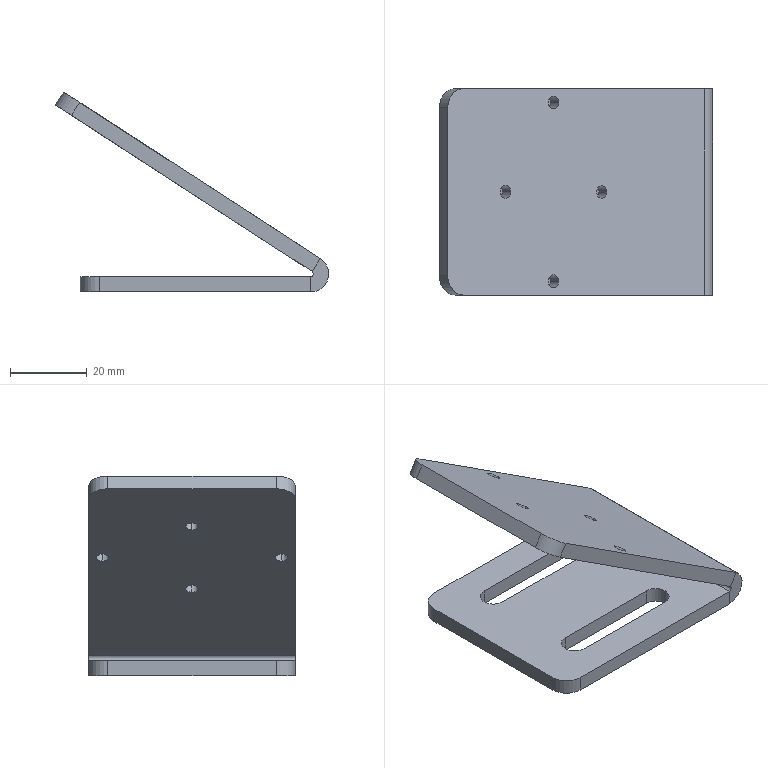Component | SolidWorks | AdjustmentPlate-1 | 1 solid | 34 faces | box 71.44 x 54 x 52.29 mm | volume 29585 mm3 | cylinder 18 | plane 16 | commonest cylinder face diameters 3.3 x8 7 x4 10 x4 9.473 x1 1.473 x1
STEP:
#1=CARTESIAN_POINT('',(2.616,-0.009211,10.905));
#2=VERTEX_POINT('',#1);
#3=CARTESIAN_POINT('',(2.507,-0.009211,10.976));
#4=VERTEX_POINT('',#3);
#5=CARTESIAN_POINT('',(2.562,-0.009211,10.941));
#6=DIRECTION('',(-0.5446,0.,-0.8387));
#7=DIRECTION('',(-0.8387,0.,0.5446));
#8=AXIS2_PLACEMENT_3D('',#5,#6,#7);
#9=CIRCLE('',#8,0.06496);
#10=EDGE_CURVE('',#2,#4,#9,.T.);
#11=ORIENTED_EDGE('',*,*,#10,.T.);
#12=CARTESIAN_POINT('',(2.593,-0.009211,11.108));
#13=VERTEX_POINT('',#12);
#14=CARTESIAN_POINT('',(2.593,-0.009211,11.108));
#15=DIRECTION('',(0.5446,-0.,0.8387));
#16=VECTOR('',#15,39.37);
#17=LINE('',#14,#16);
#18=EDGE_CURVE('',#4,#13,#17,.T.);
#19=ORIENTED_EDGE('',*,*,#18,.T.);
#20=CARTESIAN_POINT('',(2.702,-0.009211,11.037));
#21=VERTEX_POINT('',#20);
#22=CARTESIAN_POINT('',(2.647,-0.009211,11.073));
#23=DIRECTION('',(0.5446,-0.,0.8387));
#24=DIRECTION('',(0.8387,-0.,-0.5446));
#25=AXIS2_PLACEMENT_3D('',#22,#23,#24);
#26=CIRCLE('',#25,0.06496);
#27=EDGE_CURVE('',#13,#21,#26,.T.);
#28=ORIENTED_EDGE('',*,*,#27,.T.);
#29=CARTESIAN_POINT('',(2.702,-0.009211,11.037));
#30=DIRECTION('',(0.5446,-0.,0.8387));
#31=VECTOR('',#30,39.37);
#32=LINE('',#29,#31);
#33=EDGE_CURVE('',#2,#21,#32,.T.);
#34=ORIENTED_EDGE('',*,*,#33,.F.);
#35=EDGE_LOOP('',(#11,#19,#28,#34));
#36=FACE_OUTER_BOUND('',#35,.T.);
#37=CARTESIAN_POINT('',(2.647,-0.009211,11.073));
#38=DIRECTION('',(0.5446,-0.,0.8387));
#39=DIRECTION('',(0.8387,-0.,-0.5446));
#40=AXIS2_PLACEMENT_3D('',#37,#38,#39);
#41=CYLINDRICAL_SURFACE('',#40,0.06496);
#42=ADVANCED_FACE('',(#36),#41,.F.);
#43=CARTESIAN_POINT('',(1.626,-0.009211,11.549));
#44=VERTEX_POINT('',#43);
#45=CARTESIAN_POINT('',(1.517,-0.009211,11.619));
#46=VERTEX_POINT('',#45);
#47=CARTESIAN_POINT('',(1.571,-0.009211,11.584));
#48=DIRECTION('',(-0.5446,0.,-0.8387));
#49=DIRECTION('',(-0.8387,0.,0.5446));
#50=AXIS2_PLACEMENT_3D('',#47,#48,#49);
#51=CIRCLE('',#50,0.06496);
#52=EDGE_CURVE('',#44,#46,#51,.T.);
#53=ORIENTED_EDGE('',*,*,#52,.T.);
#54=CARTESIAN_POINT('',(1.602,-0.009211,11.751));
#55=VERTEX_POINT('',#54);
#56=CARTESIAN_POINT('',(1.602,-0.009211,11.751));
#57=DIRECTION('',(0.5446,-0.,0.8387));
#58=VECTOR('',#57,39.37);
#59=LINE('',#56,#58);
#60=EDGE_CURVE('',#46,#55,#59,.T.);
#61=ORIENTED_EDGE('',*,*,#60,.T.);
#62=CARTESIAN_POINT('',(1.711,-0.009211,11.681));
#63=VERTEX_POINT('',#62);
#64=CARTESIAN_POINT('',(1.657,-0.009211,11.716));
#65=DIRECTION('',(0.5446,-0.,0.8387));
#66=DIRECTION('',(0.8387,-0.,-0.5446));
#67=AXIS2_PLACEMENT_3D('',#64,#65,#66);
#68=CIRCLE('',#67,0.06496);
#69=EDGE_CURVE('',#55,#63,#68,.T.);
#70=ORIENTED_EDGE('',*,*,#69,.T.);
#71=CARTESIAN_POINT('',(1.711,-0.009211,11.681));
#72=DIRECTION('',(0.5446,-0.,0.8387));
#73=VECTOR('',#72,39.37);
#74=LINE('',#71,#73);
#75=EDGE_CURVE('',#44,#63,#74,.T.);
#76=ORIENTED_EDGE('',*,*,#75,.F.);
#77=EDGE_LOOP('',(#53,#61,#70,#76));
#78=FACE_OUTER_BOUND('',#77,.T.);
#79=CARTESIAN_POINT('',(1.657,-0.009211,11.716));
#80=DIRECTION('',(0.5446,-0.,0.8387));
#81=DIRECTION('',(0.8387,-0.,-0.5446));
#82=AXIS2_PLACEMENT_3D('',#79,#80,#81);
#83=CYLINDRICAL_SURFACE('',#82,0.06496);
#84=ADVANCED_FACE('',(#78),#83,.F.);
#85=CARTESIAN_POINT('',(2.121,0.9101,11.227));
#86=VERTEX_POINT('',#85);
#87=CARTESIAN_POINT('',(2.012,0.9101,11.298));
#88=VERTEX_POINT('',#87);
#89=CARTESIAN_POINT('',(2.066,0.9101,11.262));
#90=DIRECTION('',(-0.5446,0.,-0.8387));
#91=DIRECTION('',(-0.8387,0.,0.5446));
#92=AXIS2_PLACEMENT_3D('',#89,#90,#91);
#93=CIRCLE('',#92,0.06496);
#94=EDGE_CURVE('',#86,#88,#93,.T.);
#95=ORIENTED_EDGE('',*,*,#94,.T.);
#96=CARTESIAN_POINT('',(2.098,0.9101,11.43));
#97=VERTEX_POINT('',#96);
#98=CARTESIAN_POINT('',(2.098,0.9101,11.43));
#99=DIRECTION('',(0.5446,-0.,0.8387));
#100=VECTOR('',#99,39.37);
#101=LINE('',#98,#100);
#102=EDGE_CURVE('',#88,#97,#101,.T.);
#103=ORIENTED_EDGE('',*,*,#102,.T.);
#104=CARTESIAN_POINT('',(2.207,0.9101,11.359));
#105=VERTEX_POINT('',#104);
#106=CARTESIAN_POINT('',(2.152,0.9101,11.394));
#107=DIRECTION('',(0.5446,-0.,0.8387));
#108=DIRECTION('',(0.8387,0.,-0.5446));
#109=AXIS2_PLACEMENT_3D('',#106,#107,#108);
#110=CIRCLE('',#109,0.06496);
#111=EDGE_CURVE('',#97,#105,#110,.T.);
#112=ORIENTED_EDGE('',*,*,#111,.T.);
#113=CARTESIAN_POINT('',(2.207,0.9101,11.359));
#114=DIRECTION('',(0.5446,-0.,0.8387));
#115=VECTOR('',#114,39.37);
#116=LINE('',#113,#115);
#117=EDGE_CURVE('',#86,#105,#116,.T.);
#118=ORIENTED_EDGE('',*,*,#117,.F.);
#119=EDGE_LOOP('',(#95,#103,#112,#118));
#120=FACE_OUTER_BOUND('',#119,.T.);
#121=CARTESIAN_POINT('',(2.152,0.9101,11.394));
#122=DIRECTION('',(0.5446,-0.,0.8387));
#123=DIRECTION('',(0.8387,0.,-0.5446));
#124=AXIS2_PLACEMENT_3D('',#121,#122,#123);
#125=CYLINDRICAL_SURFACE('',#124,0.06496);
#126=ADVANCED_FACE('',(#120),#125,.F.);
#127=CARTESIAN_POINT('',(2.121,-0.9285,11.227));
#128=VERTEX_POINT('',#127);
#129=CARTESIAN_POINT('',(2.012,-0.9285,11.298));
#130=VERTEX_POINT('',#129);
#131=CARTESIAN_POINT('',(2.066,-0.9285,11.262));
#132=DIRECTION('',(-0.5446,0.,-0.8387));
#133=DIRECTION('',(-0.8387,0.,0.5446));
#134=AXIS2_PLACEMENT_3D('',#131,#132,#133);
#135=CIRCLE('',#134,0.06496);
#136=EDGE_CURVE('',#128,#130,#135,.T.);
#137=ORIENTED_EDGE('',*,*,#136,.T.);
#138=CARTESIAN_POINT('',(2.098,-0.9285,11.43));
#139=VERTEX_POINT('',#138);
#140=CARTESIAN_POINT('',(2.098,-0.9285,11.43));
#141=DIRECTION('',(0.5446,-0.,0.8387));
#142=VECTOR('',#141,39.37);
#143=LINE('',#140,#142);
#144=EDGE_CURVE('',#130,#139,#143,.T.);
#145=ORIENTED_EDGE('',*,*,#144,.T.);
#146=CARTESIAN_POINT('',(2.207,-0.9285,11.359));
#147=VERTEX_POINT('',#146);
#148=CARTESIAN_POINT('',(2.152,-0.9285,11.394));
#149=DIRECTION('',(0.5446,-0.,0.8387));
#150=DIRECTION('',(0.8387,0.,-0.5446));
#151=AXIS2_PLACEMENT_3D('',#148,#149,#150);
#152=CIRCLE('',#151,0.06496);
#153=EDGE_CURVE('',#139,#147,#152,.T.);
#154=ORIENTED_EDGE('',*,*,#153,.T.);
#155=CARTESIAN_POINT('',(2.207,-0.9285,11.359));
#156=DIRECTION('',(0.5446,-0.,0.8387));
#157=VECTOR('',#156,39.37);
#158=LINE('',#155,#157);
#159=EDGE_CURVE('',#128,#147,#158,.T.);
#160=ORIENTED_EDGE('',*,*,#159,.F.);
#161=EDGE_LOOP('',(#137,#145,#154,#160));
#162=FACE_OUTER_BOUND('',#161,.T.);
#163=CARTESIAN_POINT('',(2.152,-0.9285,11.394));
#164=DIRECTION('',(0.5446,-0.,0.8387));
#165=DIRECTION('',(0.8387,0.,-0.5446));
#166=AXIS2_PLACEMENT_3D('',#163,#164,#165);
#167=CYLINDRICAL_SURFACE('',#166,0.06496);
#168=ADVANCED_FACE('',(#162),#167,.F.);
#169=CARTESIAN_POINT('',(3.006,0.7191,10.043));
#170=VERTEX_POINT('',#169);
#171=CARTESIAN_POINT('',(3.006,0.4435,10.043));
#172=VERTEX_POINT('',#171);
#173=CARTESIAN_POINT('',(3.006,0.5813,10.043));
#174=DIRECTION('',(-0.,-0.,-1.));
#175=DIRECTION('',(0.,1.,0.));
#176=AXIS2_PLACEMENT_3D('',#173,#174,#175);
#177=CIRCLE('',#176,0.1378);
#178=EDGE_CURVE('',#170,#172,#177,.T.);
#179=ORIENTED_EDGE('',*,*,#178,.F.);
#180=CARTESIAN_POINT('',(1.824,0.7191,10.043));
#181=VERTEX_POINT('',#180);
#182=CARTESIAN_POINT('',(2.612,0.7191,10.043));
#183=DIRECTION('',(1.,-0.,-0.));
#184=VECTOR('',#183,39.37);
#185=LINE('',#182,#184);
#186=EDGE_CURVE('',#181,#170,#185,.T.);
#187=ORIENTED_EDGE('',*,*,#186,.F.);
#188=CARTESIAN_POINT('',(1.824,0.4435,10.043));
#189=VERTEX_POINT('',#188);
#190=CARTESIAN_POINT('',(1.824,0.5813,10.043));
#191=DIRECTION('',(-0.,-0.,-1.));
#192=DIRECTION('',(0.,1.,0.));
#193=AXIS2_PLACEMENT_3D('',#190,#191,#192);
#194=CIRCLE('',#193,0.1378);
#195=EDGE_CURVE('',#189,#181,#194,.T.);
#196=ORIENTED_EDGE('',*,*,#195,.F.);
#197=CARTESIAN_POINT('',(2.612,0.4435,10.043));
#198=DIRECTION('',(-1.,0.,0.));
#199=VECTOR('',#198,39.37);
#200=LINE('',#197,#199);
#201=EDGE_CURVE('',#172,#189,#200,.T.);
#202=ORIENTED_EDGE('',*,*,#201,.F.);
#203=EDGE_LOOP('',(#179,#187,#196,#202));
#204=FACE_BOUND('',#203,.T.);
#205=CARTESIAN_POINT('',(1.824,-0.7376,10.043));
#206=VERTEX_POINT('',#205);
#207=CARTESIAN_POINT('',(3.006,-0.7376,10.043));
#208=VERTEX_POINT('',#207);
#209=CARTESIAN_POINT('',(2.612,-0.7376,10.043));
#210=DIRECTION('',(1.,-0.,-0.));
#211=VECTOR('',#210,39.37);
#212=LINE('',#209,#211);
#213=EDGE_CURVE('',#206,#208,#212,.T.);
#214=ORIENTED_EDGE('',*,*,#213,.T.);
#215=CARTESIAN_POINT('',(3.006,-0.462,10.043));
#216=VERTEX_POINT('',#215);
#217=CARTESIAN_POINT('',(3.006,-0.5998,10.043));
#218=DIRECTION('',(0.,0.,1.));
#219=DIRECTION('',(0.,1.,0.));
#220=AXIS2_PLACEMENT_3D('',#217,#218,#219);
#221=CIRCLE('',#220,0.1378);
#222=EDGE_CURVE('',#208,#216,#221,.T.);
#223=ORIENTED_EDGE('',*,*,#222,.T.);
#224=CARTESIAN_POINT('',(1.824,-0.462,10.043));
#225=VERTEX_POINT('',#224);
#226=CARTESIAN_POINT('',(2.612,-0.462,10.043));
#227=DIRECTION('',(-1.,0.,0.));
#228=VECTOR('',#227,39.37);
#229=LINE('',#226,#228);
#230=EDGE_CURVE('',#216,#225,#229,.T.);
#231=ORIENTED_EDGE('',*,*,#230,.T.);
#232=CARTESIAN_POINT('',(1.824,-0.5998,10.043));
#233=DIRECTION('',(0.,0.,1.));
#234=DIRECTION('',(0.,1.,0.));
#235=AXIS2_PLACEMENT_3D('',#232,#233,#234);
#236=CIRCLE('',#235,0.1378);
#237=EDGE_CURVE('',#225,#206,#236,.T.);
#238=ORIENTED_EDGE('',*,*,#237,.T.);
#239=EDGE_LOOP('',(#214,#223,#231,#238));
#240=FACE_BOUND('',#239,.T.);
#241=CARTESIAN_POINT('',(1.234,0.8569,10.043));
#242=VERTEX_POINT('',#241);
#243=CARTESIAN_POINT('',(1.234,-0.8754,10.043));
#244=VERTEX_POINT('',#243);
#245=CARTESIAN_POINT('',(1.234,-1.072,10.043));
#246=DIRECTION('',(-0.,-1.,0.));
#247=VECTOR('',#246,39.37);
#248=LINE('',#245,#247);
#249=EDGE_CURVE('',#242,#244,#248,.T.);
#250=ORIENTED_EDGE('',*,*,#249,.F.);
#251=CARTESIAN_POINT('',(1.431,1.054,10.043));
#252=VERTEX_POINT('',#251);
#253=CARTESIAN_POINT('',(1.431,0.8569,10.043));
#254=DIRECTION('',(-0.,-0.,-1.));
#255=DIRECTION('',(0.,1.,0.));
#256=AXIS2_PLACEMENT_3D('',#253,#254,#255);
#257=CIRCLE('',#256,0.1969);
#258=EDGE_CURVE('',#242,#252,#257,.T.);
#259=ORIENTED_EDGE('',*,*,#258,.T.);
#260=CARTESIAN_POINT('',(3.603,1.054,10.043));
#261=VERTEX_POINT('',#260);
#262=CARTESIAN_POINT('',(3.99,1.054,10.043));
#263=DIRECTION('',(-1.,0.,0.));
#264=VECTOR('',#263,39.37);
#265=LINE('',#262,#264);
#266=EDGE_CURVE('',#261,#252,#265,.T.);
#267=ORIENTED_EDGE('',*,*,#266,.F.);
#268=CARTESIAN_POINT('',(3.603,-1.072,10.043));
#269=VERTEX_POINT('',#268);
#270=CARTESIAN_POINT('',(3.603,1.054,10.043));
#271=DIRECTION('',(-0.,-1.,0.));
#272=VECTOR('',#271,39.37);
#273=LINE('',#270,#272);
#274=EDGE_CURVE('',#261,#269,#273,.T.);
#275=ORIENTED_EDGE('',*,*,#274,.T.);
#276=CARTESIAN_POINT('',(1.431,-1.072,10.043));
#277=VERTEX_POINT('',#276);
#278=CARTESIAN_POINT('',(3.99,-1.072,10.043));
#279=DIRECTION('',(1.,-0.,-0.));
#280=VECTOR('',#279,39.37);
#281=LINE('',#278,#280);
#282=EDGE_CURVE('',#277,#269,#281,.T.);
#283=ORIENTED_EDGE('',*,*,#282,.F.);
#284=CARTESIAN_POINT('',(1.431,-0.8754,10.043));
#285=DIRECTION('',(-0.,-0.,-1.));
#286=DIRECTION('',(0.,1.,0.));
#287=AXIS2_PLACEMENT_3D('',#284,#285,#286);
#288=CIRCLE('',#287,0.1969);
#289=EDGE_CURVE('',#277,#244,#288,.T.);
#290=ORIENTED_EDGE('',*,*,#289,.T.);
#291=EDGE_LOOP('',(#250,#259,#267,#275,#283,#290));
#292=FACE_OUTER_BOUND('',#291,.T.);
#293=CARTESIAN_POINT('',(2.612,-0.009211,10.043));
#294=DIRECTION('',(0.,0.,1.));
#295=DIRECTION('',(0.,1.,-0.));
#296=AXIS2_PLACEMENT_3D('',#293,#294,#295);
#297=PLANE('',#296);
#298=ADVANCED_FACE('',(#204,#240,#292),#297,.F.);
#299=CARTESIAN_POINT('',(3.006,-0.7376,10.201));
#300=VERTEX_POINT('',#299);
#301=CARTESIAN_POINT('',(3.006,-0.462,10.201));
#302=VERTEX_POINT('',#301);
#303=CARTESIAN_POINT('',(3.006,-0.5998,10.201));
#304=DIRECTION('',(0.,0.,1.));
#305=DIRECTION('',(0.,1.,0.));
#306=AXIS2_PLACEMENT_3D('',#303,#304,#305);
#307=CIRCLE('',#306,0.1378);
#308=EDGE_CURVE('',#300,#302,#307,.T.);
#309=ORIENTED_EDGE('',*,*,#308,.F.);
#310=CARTESIAN_POINT('',(1.824,-0.7376,10.201));
#311=VERTEX_POINT('',#310);
#312=CARTESIAN_POINT('',(3.006,-0.7376,10.201));
#313=DIRECTION('',(1.,-0.,-0.));
#314=VECTOR('',#313,39.37);
#315=LINE('',#312,#314);
#316=EDGE_CURVE('',#311,#300,#315,.T.);
#317=ORIENTED_EDGE('',*,*,#316,.F.);
#318=CARTESIAN_POINT('',(1.824,-0.462,10.201));
#319=VERTEX_POINT('',#318);
#320=CARTESIAN_POINT('',(1.824,-0.5998,10.201));
#321=DIRECTION('',(0.,0.,1.));
#322=DIRECTION('',(0.,1.,0.));
#323=AXIS2_PLACEMENT_3D('',#320,#321,#322);
#324=CIRCLE('',#323,0.1378);
#325=EDGE_CURVE('',#319,#311,#324,.T.);
#326=ORIENTED_EDGE('',*,*,#325,.F.);
#327=CARTESIAN_POINT('',(3.006,-0.462,10.201));
#328=DIRECTION('',(-1.,0.,0.));
#329=VECTOR('',#328,39.37);
#330=LINE('',#327,#329);
#331=EDGE_CURVE('',#302,#319,#330,.T.);
#332=ORIENTED_EDGE('',*,*,#331,.F.);
#333=EDGE_LOOP('',(#309,#317,#326,#332));
#334=FACE_BOUND('',#333,.T.);
#335=CARTESIAN_POINT('',(1.824,0.7191,10.201));
#336=VERTEX_POINT('',#335);
#337=CARTESIAN_POINT('',(3.006,0.7191,10.201));
#338=VERTEX_POINT('',#337);
#339=CARTESIAN_POINT('',(3.006,0.7191,10.201));
#340=DIRECTION('',(1.,-0.,-0.));
#341=VECTOR('',#340,39.37);
#342=LINE('',#339,#341);
#343=EDGE_CURVE('',#336,#338,#342,.T.);
#344=ORIENTED_EDGE('',*,*,#343,.T.);
#345=CARTESIAN_POINT('',(3.006,0.4435,10.201));
#346=VERTEX_POINT('',#345);
#347=CARTESIAN_POINT('',(3.006,0.5813,10.201));
#348=DIRECTION('',(-0.,-0.,-1.));
#349=DIRECTION('',(0.,-1.,0.));
#350=AXIS2_PLACEMENT_3D('',#347,#348,#349);
#351=CIRCLE('',#350,0.1378);
#352=EDGE_CURVE('',#338,#346,#351,.T.);
#353=ORIENTED_EDGE('',*,*,#352,.T.);
#354=CARTESIAN_POINT('',(1.824,0.4435,10.201));
#355=VERTEX_POINT('',#354);
#356=CARTESIAN_POINT('',(3.006,0.4435,10.201));
#357=DIRECTION('',(-1.,0.,0.));
#358=VECTOR('',#357,39.37);
#359=LINE('',#356,#358);
#360=EDGE_CURVE('',#346,#355,#359,.T.);
#361=ORIENTED_EDGE('',*,*,#360,.T.);
#362=CARTESIAN_POINT('',(1.824,0.5813,10.201));
#363=DIRECTION('',(-0.,-0.,-1.));
#364=DIRECTION('',(0.,-1.,0.));
#365=AXIS2_PLACEMENT_3D('',#362,#363,#364);
#366=CIRCLE('',#365,0.1378);
#367=EDGE_CURVE('',#355,#336,#366,.T.);
#368=ORIENTED_EDGE('',*,*,#367,.T.);
#369=EDGE_LOOP('',(#344,#353,#361,#368));
#370=FACE_BOUND('',#369,.T.);
#371=CARTESIAN_POINT('',(3.603,1.054,10.201));
#372=VERTEX_POINT('',#371);
#373=CARTESIAN_POINT('',(1.431,1.054,10.201));
#374=VERTEX_POINT('',#373);
#375=CARTESIAN_POINT('',(3.99,1.054,10.201));
#376=DIRECTION('',(-1.,0.,0.));
#377=VECTOR('',#376,39.37);
#378=LINE('',#375,#377);
#379=EDGE_CURVE('',#372,#374,#378,.T.);
#380=ORIENTED_EDGE('',*,*,#379,.T.);
#381=CARTESIAN_POINT('',(1.234,0.8569,10.201));
#382=VERTEX_POINT('',#381);
#383=CARTESIAN_POINT('',(1.431,0.8569,10.201));
#384=DIRECTION('',(0.,0.,1.));
#385=DIRECTION('',(0.,1.,0.));
#386=AXIS2_PLACEMENT_3D('',#383,#384,#385);
#387=CIRCLE('',#386,0.1969);
#388=EDGE_CURVE('',#374,#382,#387,.T.);
#389=ORIENTED_EDGE('',*,*,#388,.T.);
#390=CARTESIAN_POINT('',(1.234,-0.8754,10.201));
#391=VERTEX_POINT('',#390);
#392=CARTESIAN_POINT('',(1.234,-1.072,10.201));
#393=DIRECTION('',(-0.,-1.,0.));
#394=VECTOR('',#393,39.37);
#395=LINE('',#392,#394);
#396=EDGE_CURVE('',#382,#391,#395,.T.);
#397=ORIENTED_EDGE('',*,*,#396,.T.);
#398=CARTESIAN_POINT('',(1.431,-1.072,10.201));
#399=VERTEX_POINT('',#398);
#400=CARTESIAN_POINT('',(1.431,-0.8754,10.201));
#401=DIRECTION('',(0.,0.,1.));
#402=DIRECTION('',(0.,1.,0.));
#403=AXIS2_PLACEMENT_3D('',#400,#401,#402);
#404=CIRCLE('',#403,0.1969);
#405=EDGE_CURVE('',#391,#399,#404,.T.);
#406=ORIENTED_EDGE('',*,*,#405,.T.);
#407=CARTESIAN_POINT('',(3.603,-1.072,10.201));
#408=VERTEX_POINT('',#407);
#409=CARTESIAN_POINT('',(3.99,-1.072,10.201));
#410=DIRECTION('',(1.,-0.,-0.));
#411=VECTOR('',#410,39.37);
#412=LINE('',#409,#411);
#413=EDGE_CURVE('',#399,#408,#412,.T.);
#414=ORIENTED_EDGE('',*,*,#413,.T.);
#415=CARTESIAN_POINT('',(3.603,1.054,10.201));
#416=DIRECTION('',(-0.,-1.,0.));
#417=VECTOR('',#416,39.37);
#418=LINE('',#415,#417);
#419=EDGE_CURVE('',#372,#408,#418,.T.);
#420=ORIENTED_EDGE('',*,*,#419,.F.);
#421=EDGE_LOOP('',(#380,#389,#397,#406,#414,#420));
#422=FACE_OUTER_BOUND('',#421,.T.);
#423=CARTESIAN_POINT('',(2.612,-0.009211,10.201));
#424=DIRECTION('',(0.,0.,1.));
#425=DIRECTION('',(0.,1.,-0.));
#426=AXIS2_PLACEMENT_3D('',#423,#424,#425);
#427=PLANE('',#426);
#428=ADVANCED_FACE('',(#334,#370,#422),#427,.T.);
#429=ORIENTED_EDGE('',*,*,#266,.T.);
#430=CARTESIAN_POINT('',(1.431,1.054,10.043));
#431=DIRECTION('',(0.,0.,1.));
#432=VECTOR('',#431,39.37);
#433=LINE('',#430,#432);
#434=EDGE_CURVE('',#252,#374,#433,.T.);
#435=ORIENTED_EDGE('',*,*,#434,.T.);
#436=ORIENTED_EDGE('',*,*,#379,.F.);
#437=CARTESIAN_POINT('',(3.603,1.054,10.201));
#438=DIRECTION('',(-0.,-0.,-1.));
#439=VECTOR('',#438,39.37);
#440=LINE('',#437,#439);
#441=EDGE_CURVE('',#372,#261,#440,.T.);
#442=ORIENTED_EDGE('',*,*,#441,.T.);
#443=EDGE_LOOP('',(#429,#435,#436,#442));
#444=FACE_OUTER_BOUND('',#443,.T.);
#445=CARTESIAN_POINT('',(3.99,1.054,10.043));
#446=DIRECTION('',(0.,1.,-0.));
#447=DIRECTION('',(-1.,0.,0.));
#448=AXIS2_PLACEMENT_3D('',#445,#446,#447);
#449=PLANE('',#448);
#450=ADVANCED_FACE('',(#444),#449,.T.);
#451=ORIENTED_EDGE('',*,*,#396,.F.);
#452=CARTESIAN_POINT('',(1.234,0.8569,10.043));
#453=DIRECTION('',(-0.,-0.,-1.));
#454=VECTOR('',#453,39.37);
#455=LINE('',#452,#454);
#456=EDGE_CURVE('',#382,#242,#455,.T.);
#457=ORIENTED_EDGE('',*,*,#456,.T.);
#458=ORIENTED_EDGE('',*,*,#249,.T.);
#459=CARTESIAN_POINT('',(1.234,-0.8754,10.043));
#460=DIRECTION('',(0.,0.,1.));
#461=VECTOR('',#460,39.37);
#462=LINE('',#459,#461);
#463=EDGE_CURVE('',#244,#391,#462,.T.);
#464=ORIENTED_EDGE('',*,*,#463,.T.);
#465=EDGE_LOOP('',(#451,#457,#458,#464));
#466=FACE_OUTER_BOUND('',#465,.T.);
#467=CARTESIAN_POINT('',(1.234,-1.072,10.043));
#468=DIRECTION('',(-1.,0.,0.));
#469=DIRECTION('',(-0.,-1.,0.));
#470=AXIS2_PLACEMENT_3D('',#467,#468,#469);
#471=PLANE('',#470);
#472=ADVANCED_FACE('',(#466),#471,.T.);
#473=ORIENTED_EDGE('',*,*,#413,.F.);
#474=CARTESIAN_POINT('',(1.431,-1.072,10.043));
#475=DIRECTION('',(-0.,-0.,-1.));
#476=VECTOR('',#475,39.37);
#477=LINE('',#474,#476);
#478=EDGE_CURVE('',#399,#277,#477,.T.);
#479=ORIENTED_EDGE('',*,*,#478,.T.);
#480=ORIENTED_EDGE('',*,*,#282,.T.);
#481=CARTESIAN_POINT('',(3.603,-1.072,10.201));
#482=DIRECTION('',(-0.,-0.,-1.));
#483=VECTOR('',#482,39.37);
#484=LINE('',#481,#483);
#485=EDGE_CURVE('',#408,#269,#484,.T.);
#486=ORIENTED_EDGE('',*,*,#485,.F.);
#487=EDGE_LOOP('',(#473,#479,#480,#486));
#488=FACE_OUTER_BOUND('',#487,.T.);
#489=CARTESIAN_POINT('',(3.99,-1.072,10.043));
#490=DIRECTION('',(-0.,-1.,0.));
#491=DIRECTION('',(1.,-0.,-0.));
#492=AXIS2_PLACEMENT_3D('',#489,#490,#491);
#493=PLANE('',#492);
#494=ADVANCED_FACE('',(#488),#493,.T.);
#495=CARTESIAN_POINT('',(3.006,-0.7376,9.807));
#496=DIRECTION('',(0.,0.,1.));
#497=VECTOR('',#496,39.37);
#498=LINE('',#495,#497);
#499=EDGE_CURVE('',#208,#300,#498,.T.);
#500=ORIENTED_EDGE('',*,*,#499,.T.);
#501=ORIENTED_EDGE('',*,*,#308,.T.);
#502=CARTESIAN_POINT('',(3.006,-0.462,9.807));
#503=DIRECTION('',(0.,0.,1.));
#504=VECTOR('',#503,39.37);
#505=LINE('',#502,#504);
#506=EDGE_CURVE('',#216,#302,#505,.T.);
#507=ORIENTED_EDGE('',*,*,#506,.F.);
#508=ORIENTED_EDGE('',*,*,#222,.F.);
#509=EDGE_LOOP('',(#500,#501,#507,#508));
#510=FACE_OUTER_BOUND('',#509,.T.);
#511=CARTESIAN_POINT('',(3.006,-0.5998,9.807));
#512=DIRECTION('',(0.,0.,1.));
#513=DIRECTION('',(0.,1.,0.));
#514=AXIS2_PLACEMENT_3D('',#511,#512,#513);
#515=CYLINDRICAL_SURFACE('',#514,0.1378);
#516=ADVANCED_FACE('',(#510),#515,.F.);
#517=CARTESIAN_POINT('',(1.824,-0.7376,9.807));
#518=DIRECTION('',(0.,0.,1.));
#519=VECTOR('',#518,39.37);
#520=LINE('',#517,#519);
#521=EDGE_CURVE('',#206,#311,#520,.T.);
#522=ORIENTED_EDGE('',*,*,#521,.T.);
#523=ORIENTED_EDGE('',*,*,#316,.T.);
#524=ORIENTED_EDGE('',*,*,#499,.F.);
#525=ORIENTED_EDGE('',*,*,#213,.F.);
#526=EDGE_LOOP('',(#522,#523,#524,#525));
#527=FACE_OUTER_BOUND('',#526,.T.);
#528=CARTESIAN_POINT('',(3.006,-0.7376,9.807));
#529=DIRECTION('',(-0.,-1.,0.));
#530=DIRECTION('',(1.,-0.,-0.));
#531=AXIS2_PLACEMENT_3D('',#528,#529,#530);
#532=PLANE('',#531);
#533=ADVANCED_FACE('',(#527),#532,.F.);
#534=CARTESIAN_POINT('',(1.824,-0.462,9.807));
#535=DIRECTION('',(0.,0.,1.));
#536=VECTOR('',#535,39.37);
#537=LINE('',#534,#536);
#538=EDGE_CURVE('',#225,#319,#537,.T.);
#539=ORIENTED_EDGE('',*,*,#538,.T.);
#540=ORIENTED_EDGE('',*,*,#325,.T.);
#541=ORIENTED_EDGE('',*,*,#521,.F.);
#542=ORIENTED_EDGE('',*,*,#237,.F.);
#543=EDGE_LOOP('',(#539,#540,#541,#542));
#544=FACE_OUTER_BOUND('',#543,.T.);
#545=CARTESIAN_POINT('',(1.824,-0.5998,9.807));
#546=DIRECTION('',(0.,0.,1.));
#547=DIRECTION('',(0.,1.,0.));
#548=AXIS2_PLACEMENT_3D('',#545,#546,#547);
#549=CYLINDRICAL_SURFACE('',#548,0.1378);
#550=ADVANCED_FACE('',(#544),#549,.F.);
#551=ORIENTED_EDGE('',*,*,#506,.T.);
#552=ORIENTED_EDGE('',*,*,#331,.T.);
#553=ORIENTED_EDGE('',*,*,#538,.F.);
#554=ORIENTED_EDGE('',*,*,#230,.F.);
#555=EDGE_LOOP('',(#551,#552,#553,#554));
#556=FACE_OUTER_BOUND('',#555,.T.);
#557=CARTESIAN_POINT('',(3.006,-0.462,9.807));
#558=DIRECTION('',(0.,1.,-0.));
#559=DIRECTION('',(-1.,0.,0.));
#560=AXIS2_PLACEMENT_3D('',#557,#558,#559);
#561=PLANE('',#560);
#562=ADVANCED_FACE('',(#556),#561,.F.);
#563=ORIENTED_EDGE('',*,*,#178,.T.);
#564=CARTESIAN_POINT('',(3.006,0.4435,9.807));
#565=DIRECTION('',(0.,0.,1.));
#566=VECTOR('',#565,39.37);
#567=LINE('',#564,#566);
#568=EDGE_CURVE('',#172,#346,#567,.T.);
#569=ORIENTED_EDGE('',*,*,#568,.T.);
#570=ORIENTED_EDGE('',*,*,#352,.F.);
#571=CARTESIAN_POINT('',(3.006,0.7191,9.807));
#572=DIRECTION('',(0.,0.,1.));
#573=VECTOR('',#572,39.37);
#574=LINE('',#571,#573);
#575=EDGE_CURVE('',#170,#338,#574,.T.);
#576=ORIENTED_EDGE('',*,*,#575,.F.);
#577=EDGE_LOOP('',(#563,#569,#570,#576));
#578=FACE_OUTER_BOUND('',#577,.T.);
#579=CARTESIAN_POINT('',(3.006,0.5813,9.807));
#580=DIRECTION('',(0.,0.,1.));
#581=DIRECTION('',(0.,1.,0.));
#582=AXIS2_PLACEMENT_3D('',#579,#580,#581);
#583=CYLINDRICAL_SURFACE('',#582,0.1378);
#584=ADVANCED_FACE('',(#578),#583,.F.);
#585=ORIENTED_EDGE('',*,*,#201,.T.);
#586=CARTESIAN_POINT('',(1.824,0.4435,9.807));
#587=DIRECTION('',(0.,0.,1.));
#588=VECTOR('',#587,39.37);
#589=LINE('',#586,#588);
#590=EDGE_CURVE('',#189,#355,#589,.T.);
#591=ORIENTED_EDGE('',*,*,#590,.T.);
#592=ORIENTED_EDGE('',*,*,#360,.F.);
#593=ORIENTED_EDGE('',*,*,#568,.F.);
#594=EDGE_LOOP('',(#585,#591,#592,#593));
#595=FACE_OUTER_BOUND('',#594,.T.);
#596=CARTESIAN_POINT('',(3.006,0.4435,9.807));
#597=DIRECTION('',(0.,1.,-0.));
#598=DIRECTION('',(-1.,0.,0.));
#599=AXIS2_PLACEMENT_3D('',#596,#597,#598);
#600=PLANE('',#599);
#601=ADVANCED_FACE('',(#595),#600,.T.);
#602=ORIENTED_EDGE('',*,*,#195,.T.);
#603=CARTESIAN_POINT('',(1.824,0.7191,9.807));
#604=DIRECTION('',(0.,0.,1.));
#605=VECTOR('',#604,39.37);
#606=LINE('',#603,#605);
#607=EDGE_CURVE('',#181,#336,#606,.T.);
#608=ORIENTED_EDGE('',*,*,#607,.T.);
#609=ORIENTED_EDGE('',*,*,#367,.F.);
#610=ORIENTED_EDGE('',*,*,#590,.F.);
#611=EDGE_LOOP('',(#602,#608,#609,#610));
#612=FACE_OUTER_BOUND('',#611,.T.);
#613=CARTESIAN_POINT('',(1.824,0.5813,9.807));
#614=DIRECTION('',(0.,0.,1.));
#615=DIRECTION('',(0.,1.,0.));
#616=AXIS2_PLACEMENT_3D('',#613,#614,#615);
#617=CYLINDRICAL_SURFACE('',#616,0.1378);
#618=ADVANCED_FACE('',(#612),#617,.F.);
#619=ORIENTED_EDGE('',*,*,#186,.T.);
#620=ORIENTED_EDGE('',*,*,#575,.T.);
#621=ORIENTED_EDGE('',*,*,#343,.F.);
#622=ORIENTED_EDGE('',*,*,#607,.F.);
#623=EDGE_LOOP('',(#619,#620,#621,#622));
#624=FACE_OUTER_BOUND('',#623,.T.);
#625=CARTESIAN_POINT('',(3.006,0.7191,9.807));
#626=DIRECTION('',(-0.,-1.,0.));
#627=DIRECTION('',(1.,-0.,-0.));
#628=AXIS2_PLACEMENT_3D('',#625,#626,#627);
#629=PLANE('',#628);
#630=ADVANCED_FACE('',(#624),#629,.T.);
#631=CARTESIAN_POINT('',(3.619,-1.072,10.254));
#632=VERTEX_POINT('',#631);
#633=CARTESIAN_POINT('',(3.704,-1.072,10.386));
#634=VERTEX_POINT('',#633);
#635=CARTESIAN_POINT('',(3.704,-1.072,10.386));
#636=DIRECTION('',(0.5446,-0.,0.8387));
#637=VECTOR('',#636,39.37);
#638=LINE('',#635,#637);
#639=EDGE_CURVE('',#632,#634,#638,.T.);
#640=ORIENTED_EDGE('',*,*,#639,.F.);
#641=CARTESIAN_POINT('',(3.603,-1.072,10.23));
#642=DIRECTION('',(-0.,-1.,0.));
#643=DIRECTION('',(0.,0.,-1.));
#644=AXIS2_PLACEMENT_3D('',#641,#642,#643);
#645=CIRCLE('',#644,0.029);
#646=EDGE_CURVE('',#408,#632,#645,.T.);
#647=ORIENTED_EDGE('',*,*,#646,.F.);
#648=ORIENTED_EDGE('',*,*,#485,.T.);
#649=CARTESIAN_POINT('',(3.603,-1.072,10.23));
#650=DIRECTION('',(-0.,-1.,0.));
#651=DIRECTION('',(0.,-0.,-1.));
#652=AXIS2_PLACEMENT_3D('',#649,#650,#651);
#653=CIRCLE('',#652,0.1865);
#654=EDGE_CURVE('',#269,#634,#653,.T.);
#655=ORIENTED_EDGE('',*,*,#654,.T.);
#656=EDGE_LOOP('',(#640,#647,#648,#655));
#657=FACE_OUTER_BOUND('',#656,.T.);
#658=CARTESIAN_POINT('',(3.603,-1.072,10.23));
#659=DIRECTION('',(-0.,-1.,0.));
#660=DIRECTION('',(0.,0.,1.));
#661=AXIS2_PLACEMENT_3D('',#658,#659,#660);
#662=PLANE('',#661);
#663=ADVANCED_FACE('',(#657),#662,.T.);
#664=CARTESIAN_POINT('',(3.619,1.054,10.254));
#665=VERTEX_POINT('',#664);
#666=CARTESIAN_POINT('',(3.603,1.054,10.23));
#667=DIRECTION('',(0.,1.,-0.));
#668=DIRECTION('',(0.,0.,-1.));
#669=AXIS2_PLACEMENT_3D('',#666,#667,#668);
#670=CIRCLE('',#669,0.029);
#671=EDGE_CURVE('',#665,#372,#670,.T.);
#672=ORIENTED_EDGE('',*,*,#671,.F.);
#673=CARTESIAN_POINT('',(3.704,1.054,10.386));
#674=VERTEX_POINT('',#673);
#675=CARTESIAN_POINT('',(3.619,1.054,10.254));
#676=DIRECTION('',(0.5446,-0.,0.8387));
#677=VECTOR('',#676,39.37);
#678=LINE('',#675,#677);
#679=EDGE_CURVE('',#665,#674,#678,.T.);
#680=ORIENTED_EDGE('',*,*,#679,.T.);
#681=CARTESIAN_POINT('',(3.603,1.054,10.23));
#682=DIRECTION('',(0.,1.,-0.));
#683=DIRECTION('',(0.,-0.,-1.));
#684=AXIS2_PLACEMENT_3D('',#681,#682,#683);
#685=CIRCLE('',#684,0.1865);
#686=EDGE_CURVE('',#674,#261,#685,.T.);
#687=ORIENTED_EDGE('',*,*,#686,.T.);
#688=ORIENTED_EDGE('',*,*,#441,.F.);
#689=EDGE_LOOP('',(#672,#680,#687,#688));
#690=FACE_OUTER_BOUND('',#689,.T.);
#691=CARTESIAN_POINT('',(3.603,1.054,10.23));
#692=DIRECTION('',(-0.,-1.,0.));
#693=DIRECTION('',(0.,0.,1.));
#694=AXIS2_PLACEMENT_3D('',#691,#692,#693);
#695=PLANE('',#694);
#696=ADVANCED_FACE('',(#690),#695,.F.);
#697=ORIENTED_EDGE('',*,*,#274,.F.);
#698=ORIENTED_EDGE('',*,*,#686,.F.);
#699=CARTESIAN_POINT('',(3.704,-1.072,10.386));
#700=DIRECTION('',(-0.,-1.,0.));
#701=VECTOR('',#700,39.37);
#702=LINE('',#699,#701);
#703=EDGE_CURVE('',#674,#634,#702,.T.);
#704=ORIENTED_EDGE('',*,*,#703,.T.);
#705=ORIENTED_EDGE('',*,*,#654,.F.);
#706=EDGE_LOOP('',(#697,#698,#704,#705));
#707=FACE_OUTER_BOUND('',#706,.T.);
#708=CARTESIAN_POINT('',(3.603,1.054,10.23));
#709=DIRECTION('',(0.,1.,-0.));
#710=DIRECTION('',(0.5446,0.,0.8387));
#711=AXIS2_PLACEMENT_3D('',#708,#709,#710);
#712=CYLINDRICAL_SURFACE('',#711,0.1865);
#713=ADVANCED_FACE('',(#707),#712,.T.);
#714=ORIENTED_EDGE('',*,*,#419,.T.);
#715=ORIENTED_EDGE('',*,*,#646,.T.);
#716=CARTESIAN_POINT('',(3.619,-1.072,10.254));
#717=DIRECTION('',(0.,1.,-0.));
#718=VECTOR('',#717,39.37);
#719=LINE('',#716,#718);
#720=EDGE_CURVE('',#632,#665,#719,.T.);
#721=ORIENTED_EDGE('',*,*,#720,.T.);
#722=ORIENTED_EDGE('',*,*,#671,.T.);
#723=EDGE_LOOP('',(#714,#715,#721,#722));
#724=FACE_OUTER_BOUND('',#723,.T.);
#725=CARTESIAN_POINT('',(3.603,1.054,10.23));
#726=DIRECTION('',(0.,1.,-0.));
#727=DIRECTION('',(0.5446,0.,0.8387));
#728=AXIS2_PLACEMENT_3D('',#725,#726,#727);
#729=CYLINDRICAL_SURFACE('',#728,0.029);
#730=ADVANCED_FACE('',(#724),#729,.F.);
#731=CARTESIAN_POINT('',(1.228,-1.072,11.995));
#732=VERTEX_POINT('',#731);
#733=CARTESIAN_POINT('',(2.817,-1.072,10.962));
#734=DIRECTION('',(0.8387,-0.,-0.5446));
#735=VECTOR('',#734,39.37);
#736=LINE('',#733,#735);
#737=EDGE_CURVE('',#732,#634,#736,.T.);
#738=ORIENTED_EDGE('',*,*,#737,.F.);
#739=CARTESIAN_POINT('',(1.142,-1.072,11.863));
#740=VERTEX_POINT('',#739);
#741=CARTESIAN_POINT('',(1.228,-1.072,11.995));
#742=DIRECTION('',(-0.5446,0.,-0.8387));
#743=VECTOR('',#742,39.37);
#744=LINE('',#741,#743);
#745=EDGE_CURVE('',#732,#740,#744,.T.);
#746=ORIENTED_EDGE('',*,*,#745,.T.);
#747=CARTESIAN_POINT('',(3.701,-1.072,10.201));
#748=DIRECTION('',(0.8387,-0.,-0.5446));
#749=VECTOR('',#748,39.37);
#750=LINE('',#747,#749);
#751=EDGE_CURVE('',#740,#632,#750,.T.);
#752=ORIENTED_EDGE('',*,*,#751,.T.);
#753=ORIENTED_EDGE('',*,*,#639,.T.);
#754=EDGE_LOOP('',(#738,#746,#752,#753));
#755=FACE_OUTER_BOUND('',#754,.T.);
#756=CARTESIAN_POINT('',(3.786,-1.072,10.333));
#757=DIRECTION('',(0.,1.,-0.));
#758=DIRECTION('',(-0.,-0.,-1.));
#759=AXIS2_PLACEMENT_3D('',#756,#757,#758);
#760=PLANE('',#759);
#761=ADVANCED_FACE('',(#755),#760,.F.);
#762=CARTESIAN_POINT('',(1.142,1.054,11.863));
#763=VERTEX_POINT('',#762);
#764=CARTESIAN_POINT('',(0.9767,1.054,11.97));
#765=DIRECTION('',(-0.8387,0.,0.5446));
#766=VECTOR('',#765,39.37);
#767=LINE('',#764,#766);
#768=EDGE_CURVE('',#665,#763,#767,.T.);
#769=ORIENTED_EDGE('',*,*,#768,.T.);
#770=CARTESIAN_POINT('',(1.228,1.054,11.995));
#771=VERTEX_POINT('',#770);
#772=CARTESIAN_POINT('',(1.228,1.054,11.995));
#773=DIRECTION('',(0.5446,-0.,0.8387));
#774=VECTOR('',#773,39.37);
#775=LINE('',#772,#774);
#776=EDGE_CURVE('',#763,#771,#775,.T.);
#777=ORIENTED_EDGE('',*,*,#776,.T.);
#778=CARTESIAN_POINT('',(2.817,1.054,10.962));
#779=DIRECTION('',(-0.8387,0.,0.5446));
#780=VECTOR('',#779,39.37);
#781=LINE('',#778,#780);
#782=EDGE_CURVE('',#674,#771,#781,.T.);
#783=ORIENTED_EDGE('',*,*,#782,.F.);
#784=ORIENTED_EDGE('',*,*,#679,.F.);
#785=EDGE_LOOP('',(#769,#777,#783,#784));
#786=FACE_OUTER_BOUND('',#785,.T.);
#787=CARTESIAN_POINT('',(1.062,1.054,12.102));
#788=DIRECTION('',(-0.,-1.,-0.));
#789=DIRECTION('',(1.,-0.,-0.));
#790=AXIS2_PLACEMENT_3D('',#787,#788,#789);
#791=PLANE('',#790);
#792=ADVANCED_FACE('',(#786),#791,.F.);
#793=CARTESIAN_POINT('',(2.647,-0.009211,11.073));
#794=DIRECTION('',(0.5446,-0.,0.8387));
#795=DIRECTION('',(0.8387,-0.,-0.5446));
#796=AXIS2_PLACEMENT_3D('',#793,#794,#795);
#797=CIRCLE('',#796,0.06496);
#798=EDGE_CURVE('',#21,#13,#797,.T.);
#799=ORIENTED_EDGE('',*,*,#798,.F.);
#800=ORIENTED_EDGE('',*,*,#27,.F.);
#801=EDGE_LOOP('',(#799,#800));
#802=FACE_BOUND('',#801,.T.);
#803=CARTESIAN_POINT('',(1.657,-0.009211,11.716));
#804=DIRECTION('',(0.5446,-0.,0.8387));
#805=DIRECTION('',(0.8387,-0.,-0.5446));
#806=AXIS2_PLACEMENT_3D('',#803,#804,#805);
#807=CIRCLE('',#806,0.06496);
#808=EDGE_CURVE('',#63,#55,#807,.T.);
#809=ORIENTED_EDGE('',*,*,#808,.F.);
#810=ORIENTED_EDGE('',*,*,#69,.F.);
#811=EDGE_LOOP('',(#809,#810));
#812=FACE_BOUND('',#811,.T.);
#813=CARTESIAN_POINT('',(2.152,0.9101,11.394));
#814=DIRECTION('',(0.5446,-0.,0.8387));
#815=DIRECTION('',(0.8387,0.,-0.5446));
#816=AXIS2_PLACEMENT_3D('',#813,#814,#815);
#817=CIRCLE('',#816,0.06496);
#818=EDGE_CURVE('',#105,#97,#817,.T.);
#819=ORIENTED_EDGE('',*,*,#818,.F.);
#820=ORIENTED_EDGE('',*,*,#111,.F.);
#821=EDGE_LOOP('',(#819,#820));
#822=FACE_BOUND('',#821,.T.);
#823=CARTESIAN_POINT('',(2.152,-0.9285,11.394));
#824=DIRECTION('',(0.5446,-0.,0.8387));
#825=DIRECTION('',(0.8387,0.,-0.5446));
#826=AXIS2_PLACEMENT_3D('',#823,#824,#825);
#827=CIRCLE('',#826,0.06496);
#828=EDGE_CURVE('',#147,#139,#827,.T.);
#829=ORIENTED_EDGE('',*,*,#828,.F.);
#830=ORIENTED_EDGE('',*,*,#153,.F.);
#831=EDGE_LOOP('',(#829,#830));
#832=FACE_BOUND('',#831,.T.);
#833=CARTESIAN_POINT('',(1.062,0.8569,12.102));
#834=VERTEX_POINT('',#833);
#835=CARTESIAN_POINT('',(1.062,-0.8754,12.102));
#836=VERTEX_POINT('',#835);
#837=CARTESIAN_POINT('',(1.062,-0.009211,12.102));
#838=DIRECTION('',(-0.,-1.,0.));
#839=VECTOR('',#838,39.37);
#840=LINE('',#837,#839);
#841=EDGE_CURVE('',#834,#836,#840,.T.);
#842=ORIENTED_EDGE('',*,*,#841,.T.);
#843=CARTESIAN_POINT('',(1.228,-0.8754,11.995));
#844=DIRECTION('',(0.5446,-0.,0.8387));
#845=DIRECTION('',(-0.8387,0.,0.5446));
#846=AXIS2_PLACEMENT_3D('',#843,#844,#845);
#847=CIRCLE('',#846,0.1969);
#848=EDGE_CURVE('',#836,#732,#847,.T.);
#849=ORIENTED_EDGE('',*,*,#848,.T.);
#850=ORIENTED_EDGE('',*,*,#737,.T.);
#851=ORIENTED_EDGE('',*,*,#703,.F.);
#852=ORIENTED_EDGE('',*,*,#782,.T.);
#853=CARTESIAN_POINT('',(1.228,0.8569,11.995));
#854=DIRECTION('',(0.5446,-0.,0.8387));
#855=DIRECTION('',(-0.8387,-0.,0.5446));
#856=AXIS2_PLACEMENT_3D('',#853,#854,#855);
#857=CIRCLE('',#856,0.1969);
#858=EDGE_CURVE('',#771,#834,#857,.T.);
#859=ORIENTED_EDGE('',*,*,#858,.T.);
#860=EDGE_LOOP('',(#842,#849,#850,#851,#852,#859));
#861=FACE_OUTER_BOUND('',#860,.T.);
#862=CARTESIAN_POINT('',(2.817,-0.009211,10.962));
#863=DIRECTION('',(-0.5446,0.,-0.8387));
#864=DIRECTION('',(-0.8387,0.,0.5446));
#865=AXIS2_PLACEMENT_3D('',#862,#863,#864);
#866=PLANE('',#865);
#867=ADVANCED_FACE('',(#802,#812,#822,#832,#861),#866,.F.);
#868=ORIENTED_EDGE('',*,*,#10,.F.);
#869=CARTESIAN_POINT('',(2.562,-0.009211,10.941));
#870=DIRECTION('',(-0.5446,0.,-0.8387));
#871=DIRECTION('',(-0.8387,0.,0.5446));
#872=AXIS2_PLACEMENT_3D('',#869,#870,#871);
#873=CIRCLE('',#872,0.06496);
#874=EDGE_CURVE('',#4,#2,#873,.T.);
#875=ORIENTED_EDGE('',*,*,#874,.F.);
#876=EDGE_LOOP('',(#868,#875));
#877=FACE_BOUND('',#876,.T.);
#878=ORIENTED_EDGE('',*,*,#52,.F.);
#879=CARTESIAN_POINT('',(1.571,-0.009211,11.584));
#880=DIRECTION('',(-0.5446,0.,-0.8387));
#881=DIRECTION('',(-0.8387,0.,0.5446));
#882=AXIS2_PLACEMENT_3D('',#879,#880,#881);
#883=CIRCLE('',#882,0.06496);
#884=EDGE_CURVE('',#46,#44,#883,.T.);
#885=ORIENTED_EDGE('',*,*,#884,.F.);
#886=EDGE_LOOP('',(#878,#885));
#887=FACE_BOUND('',#886,.T.);
#888=ORIENTED_EDGE('',*,*,#94,.F.);
#889=CARTESIAN_POINT('',(2.066,0.9101,11.262));
#890=DIRECTION('',(-0.5446,0.,-0.8387));
#891=DIRECTION('',(-0.8387,0.,0.5446));
#892=AXIS2_PLACEMENT_3D('',#889,#890,#891);
#893=CIRCLE('',#892,0.06496);
#894=EDGE_CURVE('',#88,#86,#893,.T.);
#895=ORIENTED_EDGE('',*,*,#894,.F.);
#896=EDGE_LOOP('',(#888,#895));
#897=FACE_BOUND('',#896,.T.);
#898=ORIENTED_EDGE('',*,*,#136,.F.);
#899=CARTESIAN_POINT('',(2.066,-0.9285,11.262));
#900=DIRECTION('',(-0.5446,0.,-0.8387));
#901=DIRECTION('',(-0.8387,0.,0.5446));
#902=AXIS2_PLACEMENT_3D('',#899,#900,#901);
#903=CIRCLE('',#902,0.06496);
#904=EDGE_CURVE('',#130,#128,#903,.T.);
#905=ORIENTED_EDGE('',*,*,#904,.F.);
#906=EDGE_LOOP('',(#898,#905));
#907=FACE_BOUND('',#906,.T.);
#908=ORIENTED_EDGE('',*,*,#751,.F.);
#909=CARTESIAN_POINT('',(0.9767,-0.8754,11.97));
#910=VERTEX_POINT('',#909);
#911=CARTESIAN_POINT('',(1.142,-0.8754,11.863));
#912=DIRECTION('',(-0.5446,0.,-0.8387));
#913=DIRECTION('',(-0.8387,0.,0.5446));
#914=AXIS2_PLACEMENT_3D('',#911,#912,#913);
#915=CIRCLE('',#914,0.1969);
#916=EDGE_CURVE('',#740,#910,#915,.T.);
#917=ORIENTED_EDGE('',*,*,#916,.T.);
#918=CARTESIAN_POINT('',(0.9767,0.8569,11.97));
#919=VERTEX_POINT('',#918);
#920=CARTESIAN_POINT('',(0.9767,-1.072,11.97));
#921=DIRECTION('',(-0.,-1.,0.));
#922=VECTOR('',#921,39.37);
#923=LINE('',#920,#922);
#924=EDGE_CURVE('',#919,#910,#923,.T.);
#925=ORIENTED_EDGE('',*,*,#924,.F.);
#926=CARTESIAN_POINT('',(1.142,0.8569,11.863));
#927=DIRECTION('',(-0.5446,0.,-0.8387));
#928=DIRECTION('',(-0.8387,0.,0.5446));
#929=AXIS2_PLACEMENT_3D('',#926,#927,#928);
#930=CIRCLE('',#929,0.1969);
#931=EDGE_CURVE('',#919,#763,#930,.T.);
#932=ORIENTED_EDGE('',*,*,#931,.T.);
#933=ORIENTED_EDGE('',*,*,#768,.F.);
#934=ORIENTED_EDGE('',*,*,#720,.F.);
#935=EDGE_LOOP('',(#908,#917,#925,#932,#933,#934));
#936=FACE_OUTER_BOUND('',#935,.T.);
#937=CARTESIAN_POINT('',(2.731,-0.009211,10.83));
#938=DIRECTION('',(-0.5446,0.,-0.8387));
#939=DIRECTION('',(-0.8387,0.,0.5446));
#940=AXIS2_PLACEMENT_3D('',#937,#938,#939);
#941=PLANE('',#940);
#942=ADVANCED_FACE('',(#877,#887,#897,#907,#936),#941,.T.);
#943=ORIENTED_EDGE('',*,*,#924,.T.);
#944=CARTESIAN_POINT('',(1.062,-0.8754,12.102));
#945=DIRECTION('',(0.5446,-0.,0.8387));
#946=VECTOR('',#945,39.37);
#947=LINE('',#944,#946);
#948=EDGE_CURVE('',#910,#836,#947,.T.);
#949=ORIENTED_EDGE('',*,*,#948,.T.);
#950=ORIENTED_EDGE('',*,*,#841,.F.);
#951=CARTESIAN_POINT('',(1.062,0.8569,12.102));
#952=DIRECTION('',(-0.5446,0.,-0.8387));
#953=VECTOR('',#952,39.37);
#954=LINE('',#951,#953);
#955=EDGE_CURVE('',#834,#919,#954,.T.);
#956=ORIENTED_EDGE('',*,*,#955,.T.);
#957=EDGE_LOOP('',(#943,#949,#950,#956));
#958=FACE_OUTER_BOUND('',#957,.T.);
#959=CARTESIAN_POINT('',(1.062,-1.072,12.102));
#960=DIRECTION('',(0.8387,-0.,-0.5446));
#961=DIRECTION('',(-0.5446,0.,-0.8387));
#962=AXIS2_PLACEMENT_3D('',#959,#960,#961);
#963=PLANE('',#962);
#964=ADVANCED_FACE('',(#958),#963,.F.);
#965=ORIENTED_EDGE('',*,*,#258,.F.);
#966=ORIENTED_EDGE('',*,*,#456,.F.);
#967=ORIENTED_EDGE('',*,*,#388,.F.);
#968=ORIENTED_EDGE('',*,*,#434,.F.);
#969=EDGE_LOOP('',(#965,#966,#967,#968));
#970=FACE_OUTER_BOUND('',#969,.T.);
#971=CARTESIAN_POINT('',(1.431,0.8569,10.043));
#972=DIRECTION('',(0.,0.,1.));
#973=DIRECTION('',(0.,1.,0.));
#974=AXIS2_PLACEMENT_3D('',#971,#972,#973);
#975=CYLINDRICAL_SURFACE('',#974,0.1969);
#976=ADVANCED_FACE('',(#970),#975,.T.);
#977=ORIENTED_EDGE('',*,*,#289,.F.);
#978=ORIENTED_EDGE('',*,*,#478,.F.);
#979=ORIENTED_EDGE('',*,*,#405,.F.);
#980=ORIENTED_EDGE('',*,*,#463,.F.);
#981=EDGE_LOOP('',(#977,#978,#979,#980));
#982=FACE_OUTER_BOUND('',#981,.T.);
#983=CARTESIAN_POINT('',(1.431,-0.8754,10.043));
#984=DIRECTION('',(0.,0.,1.));
#985=DIRECTION('',(0.,1.,0.));
#986=AXIS2_PLACEMENT_3D('',#983,#984,#985);
#987=CYLINDRICAL_SURFACE('',#986,0.1969);
#988=ADVANCED_FACE('',(#982),#987,.T.);
#989=ORIENTED_EDGE('',*,*,#848,.F.);
#990=ORIENTED_EDGE('',*,*,#948,.F.);
#991=ORIENTED_EDGE('',*,*,#916,.F.);
#992=ORIENTED_EDGE('',*,*,#745,.F.);
#993=EDGE_LOOP('',(#989,#990,#991,#992));
#994=FACE_OUTER_BOUND('',#993,.T.);
#995=CARTESIAN_POINT('',(1.228,-0.8754,11.995));
#996=DIRECTION('',(-0.5446,0.,-0.8387));
#997=DIRECTION('',(-0.8387,0.,0.5446));
#998=AXIS2_PLACEMENT_3D('',#995,#996,#997);
#999=CYLINDRICAL_SURFACE('',#998,0.1969);
#1000=ADVANCED_FACE('',(#994),#999,.T.);
#1001=ORIENTED_EDGE('',*,*,#858,.F.);
#1002=ORIENTED_EDGE('',*,*,#776,.F.);
#1003=ORIENTED_EDGE('',*,*,#931,.F.);
#1004=ORIENTED_EDGE('',*,*,#955,.F.);
#1005=EDGE_LOOP('',(#1001,#1002,#1003,#1004));
#1006=FACE_OUTER_BOUND('',#1005,.T.);
#1007=CARTESIAN_POINT('',(1.228,0.8569,11.995));
#1008=DIRECTION('',(-0.5446,0.,-0.8387));
#1009=DIRECTION('',(-0.8387,0.,0.5446));
#1010=AXIS2_PLACEMENT_3D('',#1007,#1008,#1009);
#1011=CYLINDRICAL_SURFACE('',#1010,0.1969);
#1012=ADVANCED_FACE('',(#1006),#1011,.T.);
#1013=ORIENTED_EDGE('',*,*,#144,.F.);
#1014=ORIENTED_EDGE('',*,*,#904,.T.);
#1015=ORIENTED_EDGE('',*,*,#159,.T.);
#1016=ORIENTED_EDGE('',*,*,#828,.T.);
#1017=EDGE_LOOP('',(#1013,#1014,#1015,#1016));
#1018=FACE_OUTER_BOUND('',#1017,.T.);
#1019=CARTESIAN_POINT('',(2.152,-0.9285,11.394));
#1020=DIRECTION('',(0.5446,-0.,0.8387));
#1021=DIRECTION('',(0.8387,0.,-0.5446));
#1022=AXIS2_PLACEMENT_3D('',#1019,#1020,#1021);
#1023=CYLINDRICAL_SURFACE('',#1022,0.06496);
#1024=ADVANCED_FACE('',(#1018),#1023,.F.);
#1025=ORIENTED_EDGE('',*,*,#102,.F.);
#1026=ORIENTED_EDGE('',*,*,#894,.T.);
#1027=ORIENTED_EDGE('',*,*,#117,.T.);
#1028=ORIENTED_EDGE('',*,*,#818,.T.);
#1029=EDGE_LOOP('',(#1025,#1026,#1027,#1028));
#1030=FACE_OUTER_BOUND('',#1029,.T.);
#1031=CARTESIAN_POINT('',(2.152,0.9101,11.394));
#1032=DIRECTION('',(0.5446,-0.,0.8387));
#1033=DIRECTION('',(0.8387,0.,-0.5446));
#1034=AXIS2_PLACEMENT_3D('',#1031,#1032,#1033);
#1035=CYLINDRICAL_SURFACE('',#1034,0.06496);
#1036=ADVANCED_FACE('',(#1030),#1035,.F.);
#1037=ORIENTED_EDGE('',*,*,#60,.F.);
#1038=ORIENTED_EDGE('',*,*,#884,.T.);
#1039=ORIENTED_EDGE('',*,*,#75,.T.);
#1040=ORIENTED_EDGE('',*,*,#808,.T.);
#1041=EDGE_LOOP('',(#1037,#1038,#1039,#1040));
#1042=FACE_OUTER_BOUND('',#1041,.T.);
#1043=CARTESIAN_POINT('',(1.657,-0.009211,11.716));
#1044=DIRECTION('',(0.5446,-0.,0.8387));
#1045=DIRECTION('',(0.8387,-0.,-0.5446));
#1046=AXIS2_PLACEMENT_3D('',#1043,#1044,#1045);
#1047=CYLINDRICAL_SURFACE('',#1046,0.06496);
#1048=ADVANCED_FACE('',(#1042),#1047,.F.);
#1049=ORIENTED_EDGE('',*,*,#18,.F.);
#1050=ORIENTED_EDGE('',*,*,#874,.T.);
#1051=ORIENTED_EDGE('',*,*,#33,.T.);
#1052=ORIENTED_EDGE('',*,*,#798,.T.);
#1053=EDGE_LOOP('',(#1049,#1050,#1051,#1052));
#1054=FACE_OUTER_BOUND('',#1053,.T.);
#1055=CARTESIAN_POINT('',(2.647,-0.009211,11.073));
#1056=DIRECTION('',(0.5446,-0.,0.8387));
#1057=DIRECTION('',(0.8387,-0.,-0.5446));
#1058=AXIS2_PLACEMENT_3D('',#1055,#1056,#1057);
#1059=CYLINDRICAL_SURFACE('',#1058,0.06496);
#1060=ADVANCED_FACE('',(#1054),#1059,.F.);
#1061=CLOSED_SHELL('',(#42,#84,#126,#168,#298,#428,#450,#472,#494,#516,#533,#550,#562,#584,#601,#618,#630,#663,#696,#713,#730,#761,#792,#867,#942,#964,#976,#988,#1000,#1012,#1024,#1036,#1048,#1060));
#1062=MANIFOLD_SOLID_BREP('',#1061);
#1063=CARTESIAN_POINT('',(0.,0.,0.));
#1064=DIRECTION('',(0.,0.,1.));
#1065=DIRECTION('',(1.,0.,0.));
#1066=AXIS2_PLACEMENT_3D('',#1063,#1064,#1065);
#1067=(LENGTH_UNIT()NAMED_UNIT(*)SI_UNIT($,.METRE.));
#1068=LENGTH_MEASURE_WITH_UNIT(LENGTH_MEASURE(0.0254),#1067);
#1069=DIMENSIONAL_EXPONENTS(1.,0.,0.,0.,0.,0.,0.);
#1070=(CONVERSION_BASED_UNIT('',#1068)LENGTH_UNIT()NAMED_UNIT(#1069));
#1071=UNCERTAINTY_MEASURE_WITH_UNIT(LENGTH_MEASURE(0.00001),#1070,'','');
#1072=(NAMED_UNIT(*)PLANE_ANGLE_UNIT()SI_UNIT($,.RADIAN.));
#1073=(NAMED_UNIT(*)SI_UNIT($,.STERADIAN.)SOLID_ANGLE_UNIT());
#1074=(GEOMETRIC_REPRESENTATION_CONTEXT(3)GLOBAL_UNCERTAINTY_ASSIGNED_CONTEXT((#1071))GLOBAL_UNIT_ASSIGNED_CONTEXT((#1070,#1072,#1073))REPRESENTATION_CONTEXT('',''));
#1075=ADVANCED_BREP_SHAPE_REPRESENTATION('',(#1062,#1066),#1074);
#1076=COLOUR_RGB('',0.7922,0.8196,0.9333);
#1077=FILL_AREA_STYLE_COLOUR('',#1076);
#1078=FILL_AREA_STYLE('',(#1077));
#1079=SURFACE_STYLE_FILL_AREA(#1078);
#1080=SURFACE_SIDE_STYLE('',(#1079));
#1081=SURFACE_STYLE_USAGE(.BOTH.,#1080);
#1082=PRESENTATION_STYLE_ASSIGNMENT((#1081));
#1083=STYLED_ITEM('',(#1082),#1062);
#1084=PRESENTATION_LAYER_ASSIGNMENT('','',(#1083));
#1085=(LENGTH_UNIT()NAMED_UNIT(*)SI_UNIT($,.METRE.));
#1086=LENGTH_MEASURE_WITH_UNIT(LENGTH_MEASURE(0.0254),#1085);
#1087=DIMENSIONAL_EXPONENTS(1.,0.,0.,0.,0.,0.,0.);
#1088=(CONVERSION_BASED_UNIT('',#1086)LENGTH_UNIT()NAMED_UNIT(#1087));
#1089=UNCERTAINTY_MEASURE_WITH_UNIT(LENGTH_MEASURE(0.00001),#1088,'','');
#1090=(NAMED_UNIT(*)PLANE_ANGLE_UNIT()SI_UNIT($,.RADIAN.));
#1091=(NAMED_UNIT(*)SI_UNIT($,.STERADIAN.)SOLID_ANGLE_UNIT());
#1092=(GEOMETRIC_REPRESENTATION_CONTEXT(3)GLOBAL_UNCERTAINTY_ASSIGNED_CONTEXT((#1089))GLOBAL_UNIT_ASSIGNED_CONTEXT((#1088,#1090,#1091))REPRESENTATION_CONTEXT('',''));
#1093=MECHANICAL_DESIGN_GEOMETRIC_PRESENTATION_REPRESENTATION('',(#1083),#1092);